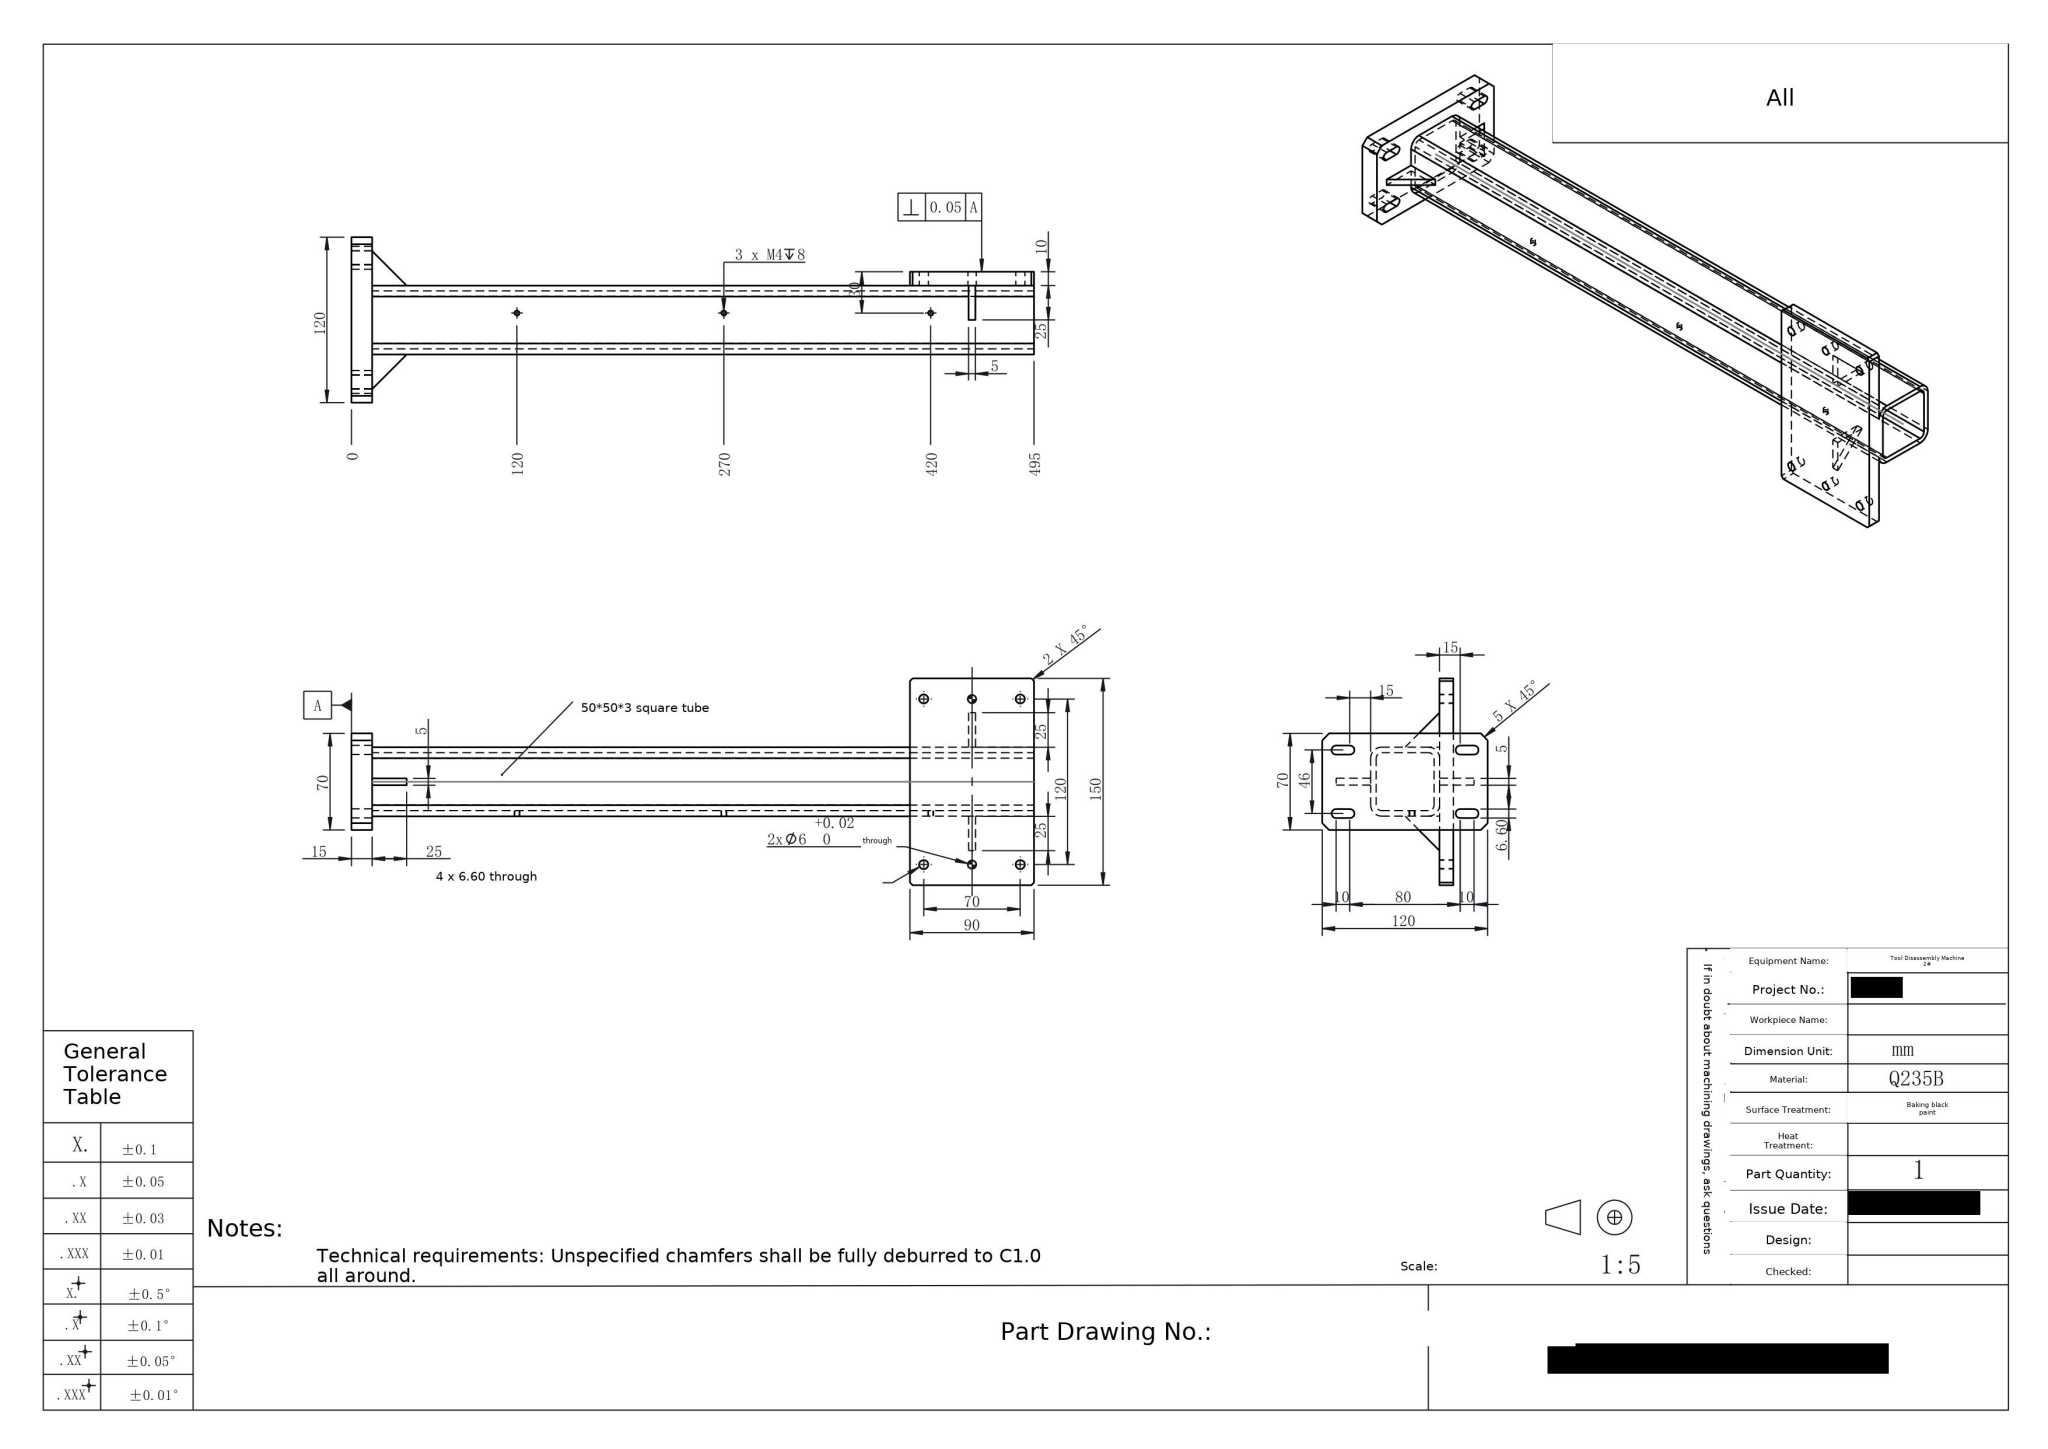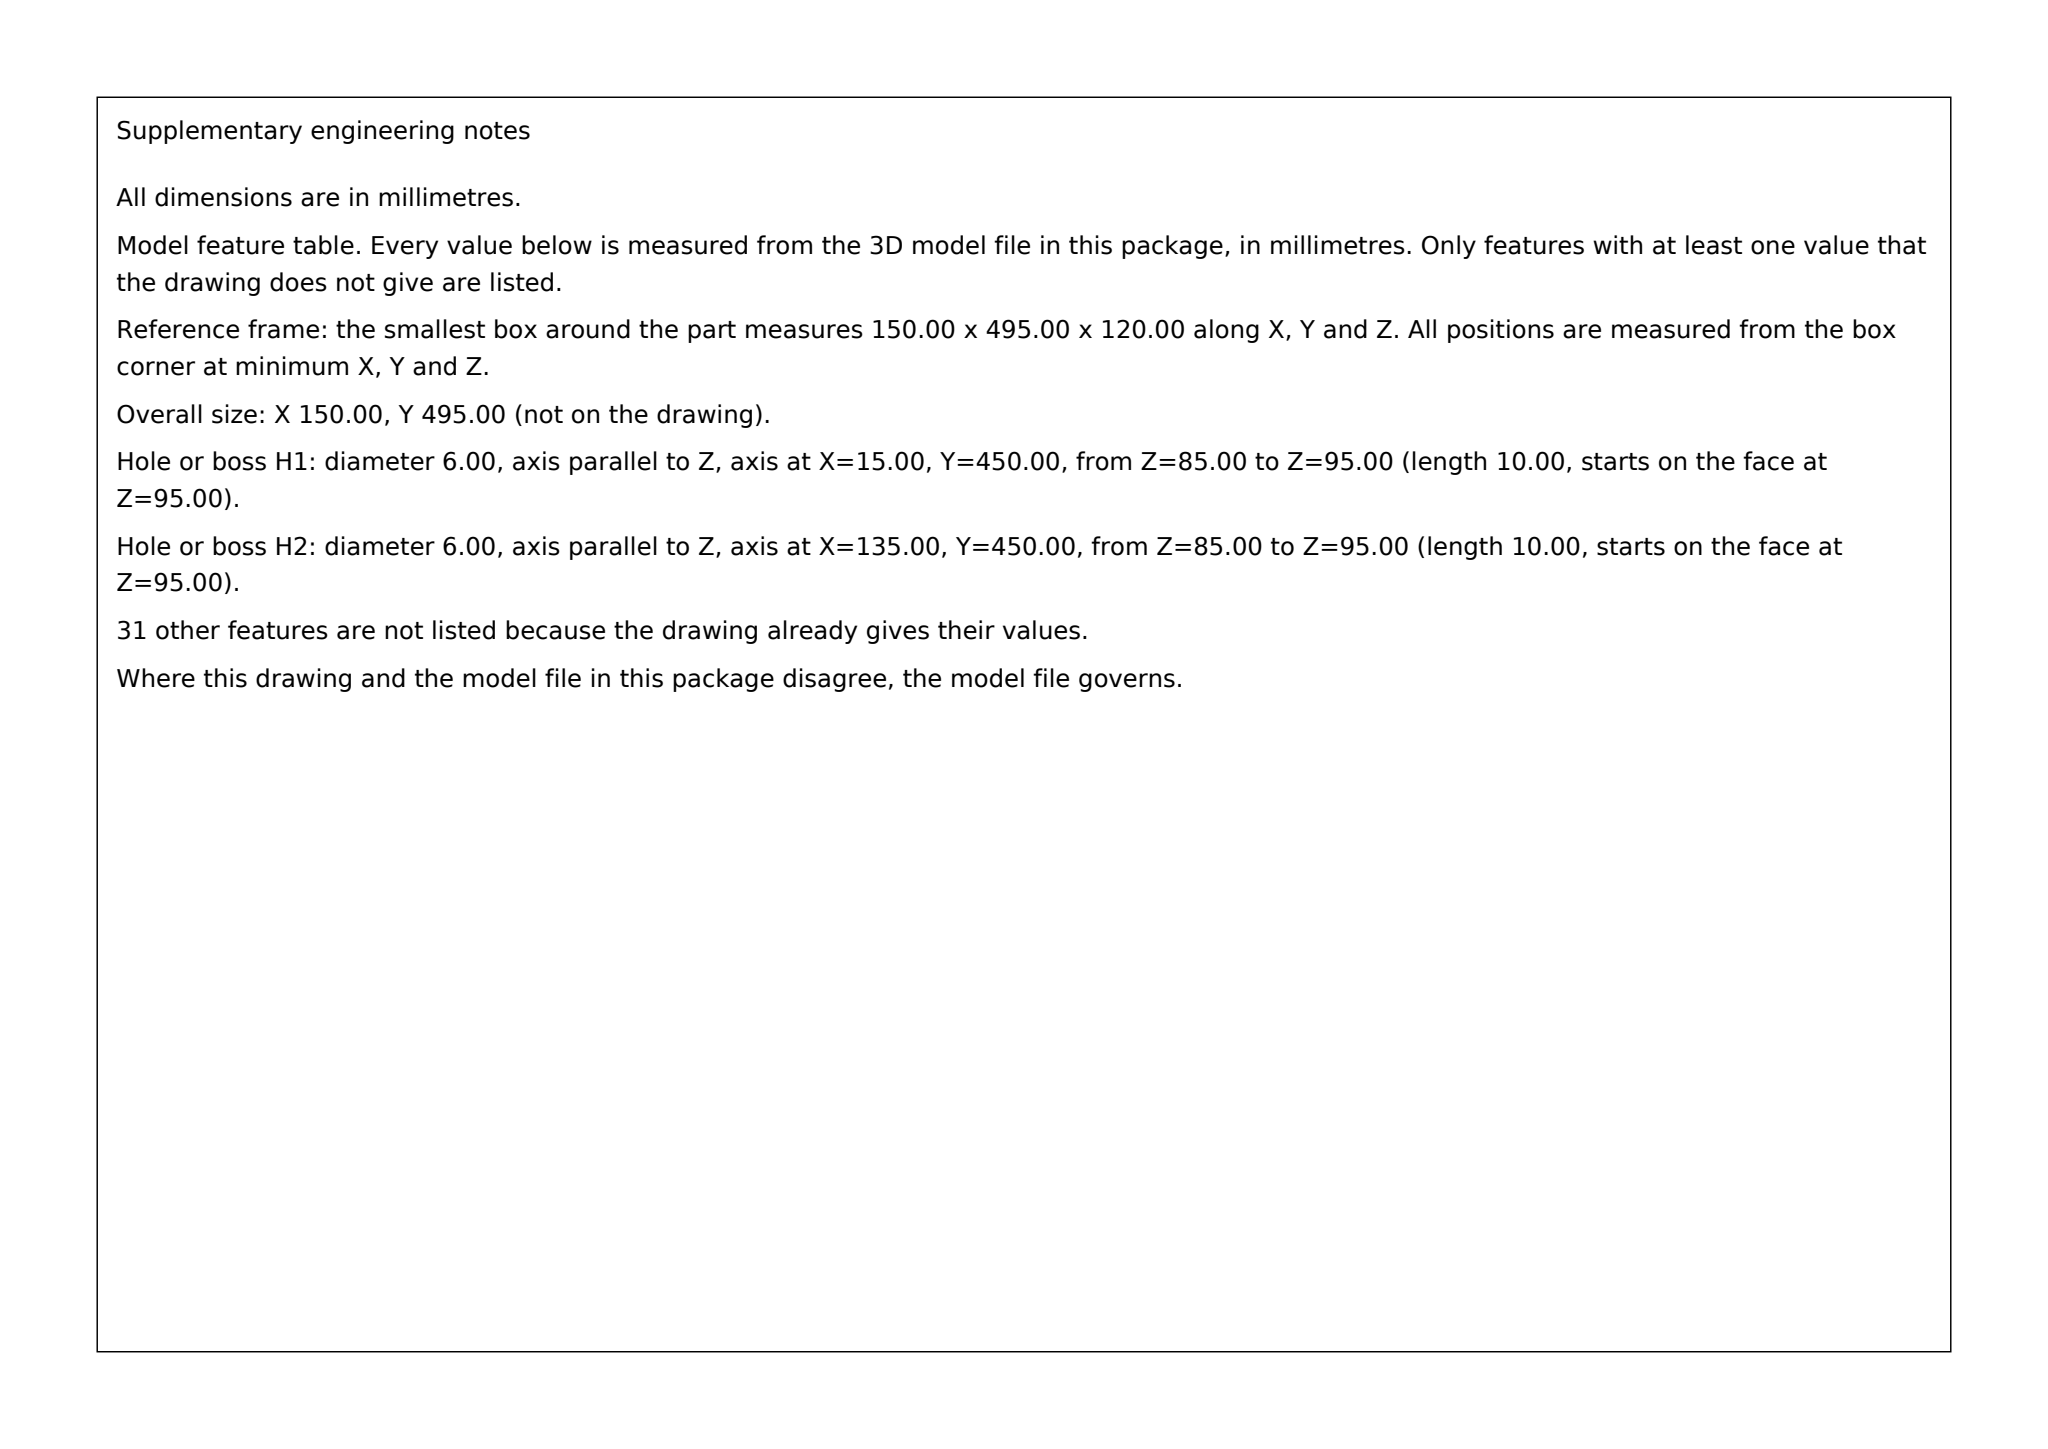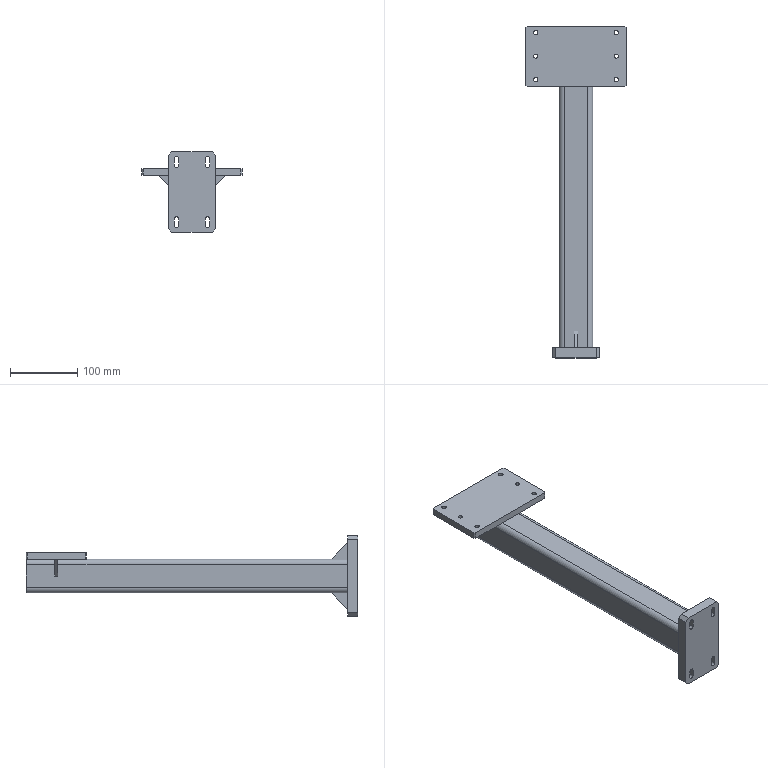Part | SolidWorks | mm | material Q235B | 1 solid | 90 faces | box 150 x 495 x 120 mm | volume 591873 mm3 | plane 52 | cylinder 38 | commonest cylinder face diameters 6.6 x20 3.3 x6 6 x4 16 x4 8 x4